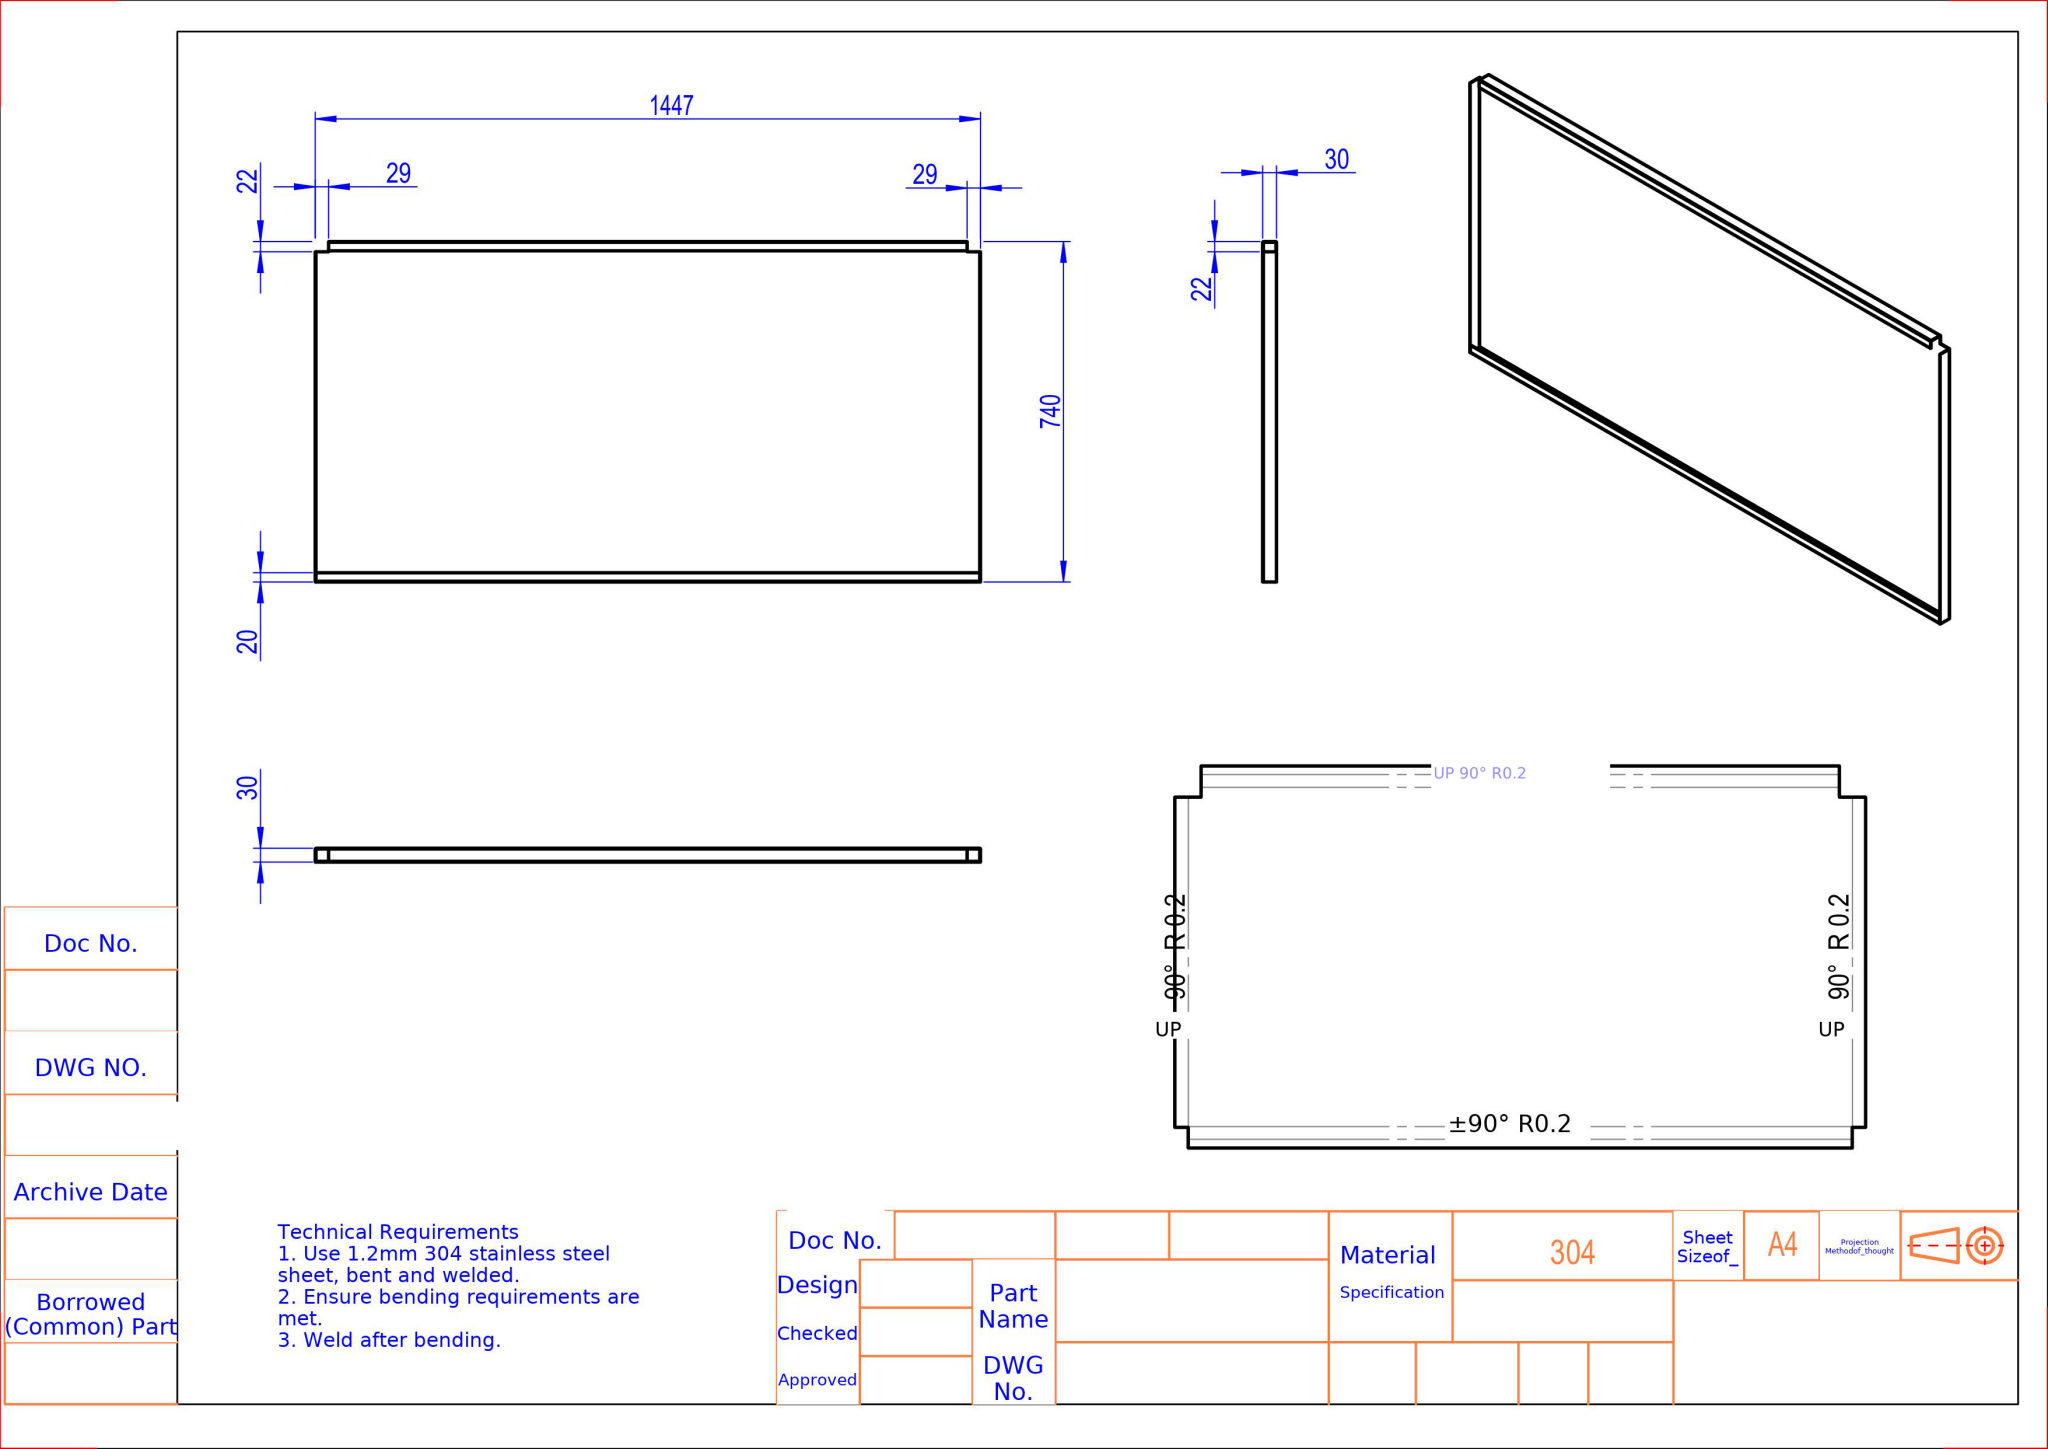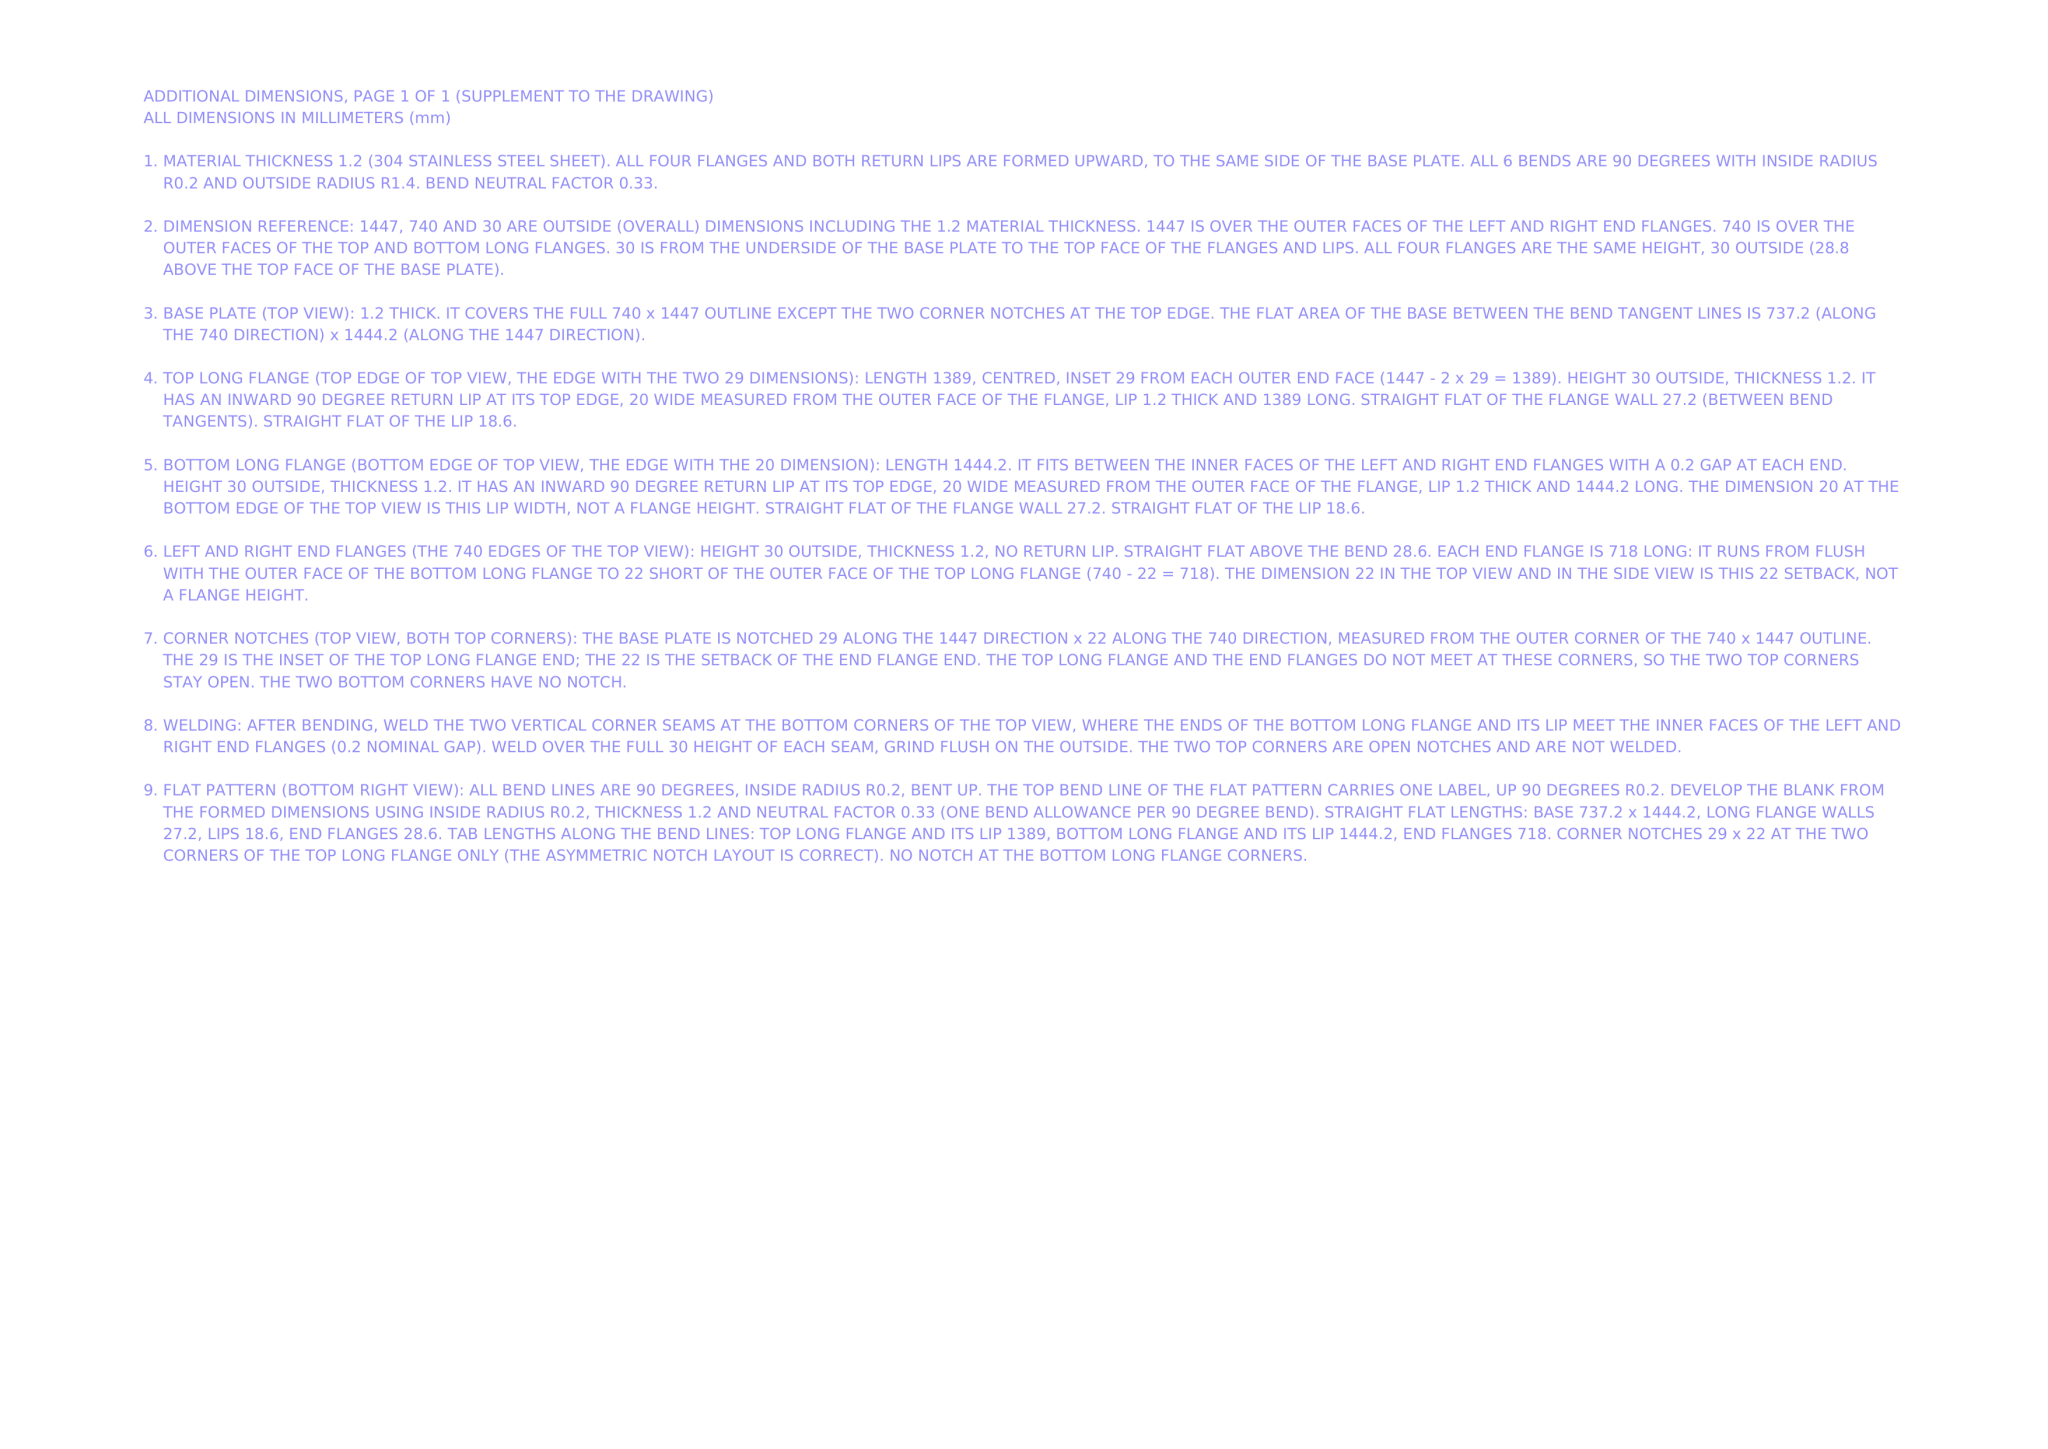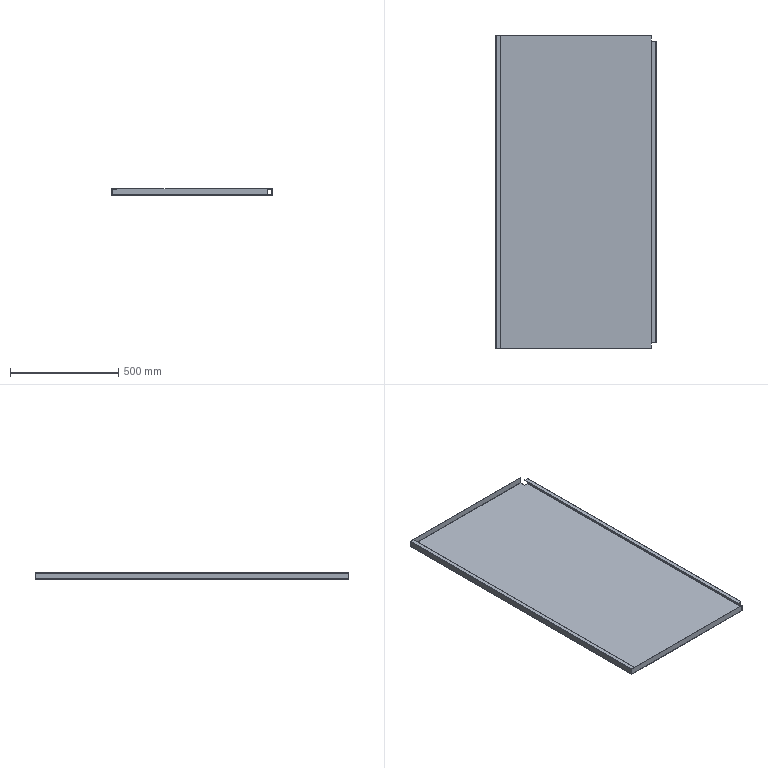Part | NX | mm | 1 solid | 60 faces | box 740 x 1447 x 30 mm | volume 1491939 mm3 | plane 48 | cylinder 12 | commonest cylinder face diameters 2.8 x6 0.4 x6